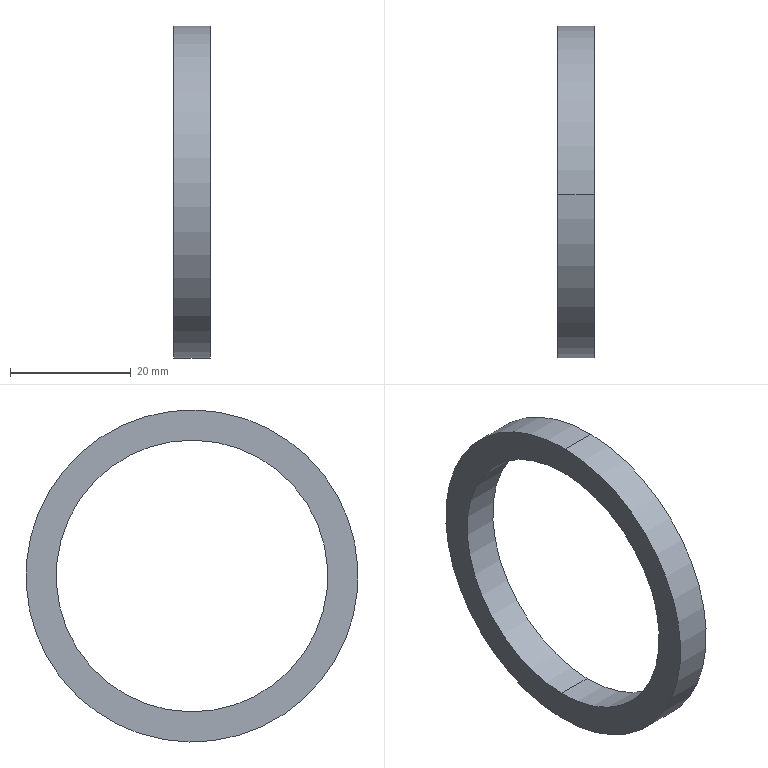Component | SolidWorks | 216InnerTubeAssembly-1_BearingSpacer1-1 | 1 solid | 6 faces | box 6 x 55 x 55 mm | volume 4712 mm3 | cylinder 4 | plane 2 | commonest cylinder face diameters 45 x2 55 x2 | material Alloy Steel
build123d program:
from build123d import *

# Parameters (mm, degrees)
MODEL_W = 5.999
MODEL_H = 5


with BuildPart() as part:
    # Model → Revolve1 (revolve)
    with BuildSketch(Plane.XY, mode=Mode.PRIVATE) as revolve1_sk:
        with Locations((2.999, 25)):
            Rectangle(MODEL_W, MODEL_H)
    revolve(revolve1_sk.sketch.rotate(Axis((0, 0, 0), (1, 0, 0)), 90), axis=Axis((0, 0, 0), (1, 0, 0)))


solid = part.part

# Placed as in the assembly
solid = solid.moved(Location((841.279, 0, 0), (0, 0, 0)))
STEP:
#1=COLOUR_RGB('',0.7922,0.8196,0.9333);
#2=FILL_AREA_STYLE_COLOUR('',#1);
#3=FILL_AREA_STYLE('',(#2));
#4=SURFACE_STYLE_FILL_AREA(#3);
#5=SURFACE_SIDE_STYLE('',(#4));
#6=SURFACE_STYLE_USAGE(.BOTH.,#5);
#7=PRESENTATION_STYLE_ASSIGNMENT((#6));
#8=CARTESIAN_POINT('',(33.357,0.01591,-0.8857));
#9=VERTEX_POINT('',#8);
#10=CARTESIAN_POINT('',(33.357,-0.01591,0.8857));
#11=VERTEX_POINT('',#10);
#12=CARTESIAN_POINT('',(33.357,-0.,0.));
#13=DIRECTION('',(-1.,-0.,0.));
#14=DIRECTION('',(0.,-0.01796,0.9998));
#15=AXIS2_PLACEMENT_3D('',#12,#13,#14);
#16=CIRCLE('',#15,0.8858);
#17=EDGE_CURVE('',#9,#11,#16,.T.);
#18=ORIENTED_EDGE('',*,*,#17,.F.);
#19=CARTESIAN_POINT('',(33.121,0.01591,-0.8857));
#20=VERTEX_POINT('',#19);
#21=CARTESIAN_POINT('',(33.121,0.01591,-0.8857));
#22=DIRECTION('',(-1.,-0.,0.));
#23=VECTOR('',#22,39.37);
#24=LINE('',#21,#23);
#25=EDGE_CURVE('',#9,#20,#24,.T.);
#26=ORIENTED_EDGE('',*,*,#25,.T.);
#27=CARTESIAN_POINT('',(33.121,-0.01591,0.8857));
#28=VERTEX_POINT('',#27);
#29=CARTESIAN_POINT('',(33.121,-0.,0.));
#30=DIRECTION('',(-1.,-0.,0.));
#31=DIRECTION('',(0.,-0.01796,0.9998));
#32=AXIS2_PLACEMENT_3D('',#29,#30,#31);
#33=CIRCLE('',#32,0.8858);
#34=EDGE_CURVE('',#20,#28,#33,.T.);
#35=ORIENTED_EDGE('',*,*,#34,.T.);
#36=CARTESIAN_POINT('',(33.121,-0.01591,0.8857));
#37=DIRECTION('',(-1.,-0.,0.));
#38=VECTOR('',#37,39.37);
#39=LINE('',#36,#38);
#40=EDGE_CURVE('',#11,#28,#39,.T.);
#41=ORIENTED_EDGE('',*,*,#40,.F.);
#42=EDGE_LOOP('',(#18,#26,#35,#41));
#43=FACE_OUTER_BOUND('',#42,.T.);
#44=CARTESIAN_POINT('',(33.121,-0.,0.));
#45=DIRECTION('',(-1.,-0.,0.));
#46=DIRECTION('',(0.,-0.01796,0.9998));
#47=AXIS2_PLACEMENT_3D('',#44,#45,#46);
#48=CYLINDRICAL_SURFACE('',#47,0.8858);
#49=ADVANCED_FACE('',(#43),#48,.F.);
#50=CARTESIAN_POINT('',(33.357,-0.01944,1.083));
#51=VERTEX_POINT('',#50);
#52=CARTESIAN_POINT('',(33.357,0.01944,-1.083));
#53=VERTEX_POINT('',#52);
#54=CARTESIAN_POINT('',(33.357,-0.,0.));
#55=DIRECTION('',(-1.,-0.,0.));
#56=DIRECTION('',(0.,-0.01796,0.9998));
#57=AXIS2_PLACEMENT_3D('',#54,#55,#56);
#58=CIRCLE('',#57,1.083);
#59=EDGE_CURVE('',#51,#53,#58,.T.);
#60=ORIENTED_EDGE('',*,*,#59,.T.);
#61=CARTESIAN_POINT('',(33.121,0.01944,-1.083));
#62=VERTEX_POINT('',#61);
#63=CARTESIAN_POINT('',(33.121,0.01944,-1.083));
#64=DIRECTION('',(-1.,-0.,0.));
#65=VECTOR('',#64,39.37);
#66=LINE('',#63,#65);
#67=EDGE_CURVE('',#53,#62,#66,.T.);
#68=ORIENTED_EDGE('',*,*,#67,.T.);
#69=CARTESIAN_POINT('',(33.121,-0.01944,1.083));
#70=VERTEX_POINT('',#69);
#71=CARTESIAN_POINT('',(33.121,-0.,0.));
#72=DIRECTION('',(-1.,-0.,0.));
#73=DIRECTION('',(0.,-0.01796,0.9998));
#74=AXIS2_PLACEMENT_3D('',#71,#72,#73);
#75=CIRCLE('',#74,1.083);
#76=EDGE_CURVE('',#70,#62,#75,.T.);
#77=ORIENTED_EDGE('',*,*,#76,.F.);
#78=CARTESIAN_POINT('',(33.121,-0.01944,1.083));
#79=DIRECTION('',(-1.,-0.,0.));
#80=VECTOR('',#79,39.37);
#81=LINE('',#78,#80);
#82=EDGE_CURVE('',#51,#70,#81,.T.);
#83=ORIENTED_EDGE('',*,*,#82,.F.);
#84=EDGE_LOOP('',(#60,#68,#77,#83));
#85=FACE_OUTER_BOUND('',#84,.T.);
#86=CARTESIAN_POINT('',(33.121,-0.,0.));
#87=DIRECTION('',(-1.,-0.,0.));
#88=DIRECTION('',(0.,-0.01796,0.9998));
#89=AXIS2_PLACEMENT_3D('',#86,#87,#88);
#90=CYLINDRICAL_SURFACE('',#89,1.083);
#91=ADVANCED_FACE('',(#85),#90,.T.);
#92=ORIENTED_EDGE('',*,*,#67,.F.);
#93=CARTESIAN_POINT('',(33.357,-0.,0.));
#94=DIRECTION('',(-1.,-0.,0.));
#95=DIRECTION('',(0.,-0.01796,0.9998));
#96=AXIS2_PLACEMENT_3D('',#93,#94,#95);
#97=CIRCLE('',#96,1.083);
#98=EDGE_CURVE('',#53,#51,#97,.T.);
#99=ORIENTED_EDGE('',*,*,#98,.T.);
#100=ORIENTED_EDGE('',*,*,#82,.T.);
#101=CARTESIAN_POINT('',(33.121,-0.,0.));
#102=DIRECTION('',(-1.,-0.,0.));
#103=DIRECTION('',(0.,-0.01796,0.9998));
#104=AXIS2_PLACEMENT_3D('',#101,#102,#103);
#105=CIRCLE('',#104,1.083);
#106=EDGE_CURVE('',#62,#70,#105,.T.);
#107=ORIENTED_EDGE('',*,*,#106,.F.);
#108=EDGE_LOOP('',(#92,#99,#100,#107));
#109=FACE_OUTER_BOUND('',#108,.T.);
#110=CARTESIAN_POINT('',(33.121,-0.,0.));
#111=DIRECTION('',(-1.,-0.,0.));
#112=DIRECTION('',(0.,-0.01796,0.9998));
#113=AXIS2_PLACEMENT_3D('',#110,#111,#112);
#114=CYLINDRICAL_SURFACE('',#113,1.083);
#115=ADVANCED_FACE('',(#109),#114,.T.);
#116=CARTESIAN_POINT('',(33.121,-0.,0.));
#117=DIRECTION('',(-1.,-0.,0.));
#118=DIRECTION('',(0.,-0.01796,0.9998));
#119=AXIS2_PLACEMENT_3D('',#116,#117,#118);
#120=CIRCLE('',#119,0.8858);
#121=EDGE_CURVE('',#28,#20,#120,.T.);
#122=ORIENTED_EDGE('',*,*,#121,.F.);
#123=ORIENTED_EDGE('',*,*,#34,.F.);
#124=EDGE_LOOP('',(#122,#123));
#125=FACE_BOUND('',#124,.T.);
#126=ORIENTED_EDGE('',*,*,#76,.T.);
#127=ORIENTED_EDGE('',*,*,#106,.T.);
#128=EDGE_LOOP('',(#126,#127));
#129=FACE_OUTER_BOUND('',#128,.T.);
#130=CARTESIAN_POINT('',(33.121,1.083,0.01944));
#131=DIRECTION('',(1.,0.,-0.));
#132=DIRECTION('',(-0.,0.01796,-0.9998));
#133=AXIS2_PLACEMENT_3D('',#130,#131,#132);
#134=PLANE('',#133);
#135=ADVANCED_FACE('',(#125,#129),#134,.F.);
#136=ORIENTED_EDGE('',*,*,#25,.F.);
#137=CARTESIAN_POINT('',(33.357,-0.,0.));
#138=DIRECTION('',(-1.,-0.,0.));
#139=DIRECTION('',(0.,-0.01796,0.9998));
#140=AXIS2_PLACEMENT_3D('',#137,#138,#139);
#141=CIRCLE('',#140,0.8858);
#142=EDGE_CURVE('',#11,#9,#141,.T.);
#143=ORIENTED_EDGE('',*,*,#142,.F.);
#144=ORIENTED_EDGE('',*,*,#40,.T.);
#145=ORIENTED_EDGE('',*,*,#121,.T.);
#146=EDGE_LOOP('',(#136,#143,#144,#145));
#147=FACE_OUTER_BOUND('',#146,.T.);
#148=CARTESIAN_POINT('',(33.121,-0.,0.));
#149=DIRECTION('',(-1.,-0.,0.));
#150=DIRECTION('',(0.,-0.01796,0.9998));
#151=AXIS2_PLACEMENT_3D('',#148,#149,#150);
#152=CYLINDRICAL_SURFACE('',#151,0.8858);
#153=ADVANCED_FACE('',(#147),#152,.F.);
#154=ORIENTED_EDGE('',*,*,#59,.F.);
#155=ORIENTED_EDGE('',*,*,#98,.F.);
#156=EDGE_LOOP('',(#154,#155));
#157=FACE_OUTER_BOUND('',#156,.T.);
#158=ORIENTED_EDGE('',*,*,#142,.T.);
#159=ORIENTED_EDGE('',*,*,#17,.T.);
#160=EDGE_LOOP('',(#158,#159));
#161=FACE_BOUND('',#160,.T.);
#162=CARTESIAN_POINT('',(33.357,0.8857,0.01591));
#163=DIRECTION('',(-1.,-0.,0.));
#164=DIRECTION('',(0.,-0.01796,0.9998));
#165=AXIS2_PLACEMENT_3D('',#162,#163,#164);
#166=PLANE('',#165);
#167=ADVANCED_FACE('',(#157,#161),#166,.F.);
#168=CLOSED_SHELL('',(#49,#91,#115,#135,#153,#167));
#169=MANIFOLD_SOLID_BREP('',#168);
#170=STYLED_ITEM('',(#7),#169);
#171=(LENGTH_UNIT()NAMED_UNIT(*)SI_UNIT($,.METRE.));
#172=LENGTH_MEASURE_WITH_UNIT(LENGTH_MEASURE(0.0254),#171);
#173=DIMENSIONAL_EXPONENTS(1.,0.,0.,0.,0.,0.,0.);
#174=(CONVERSION_BASED_UNIT('',#172)LENGTH_UNIT()NAMED_UNIT(#173));
#175=UNCERTAINTY_MEASURE_WITH_UNIT(LENGTH_MEASURE(0.00001),#174,'','');
#176=(NAMED_UNIT(*)PLANE_ANGLE_UNIT()SI_UNIT($,.RADIAN.));
#177=(NAMED_UNIT(*)SI_UNIT($,.STERADIAN.)SOLID_ANGLE_UNIT());
#178=(GEOMETRIC_REPRESENTATION_CONTEXT(3)GLOBAL_UNCERTAINTY_ASSIGNED_CONTEXT((#175))GLOBAL_UNIT_ASSIGNED_CONTEXT((#174,#176,#177))REPRESENTATION_CONTEXT('',''));
#179=MECHANICAL_DESIGN_GEOMETRIC_PRESENTATION_REPRESENTATION('',(#170),#178);
#180=CARTESIAN_POINT('',(0.,0.,0.));
#181=DIRECTION('',(0.,0.,1.));
#182=DIRECTION('',(1.,0.,0.));
#183=AXIS2_PLACEMENT_3D('',#180,#181,#182);
#184=(LENGTH_UNIT()NAMED_UNIT(*)SI_UNIT($,.METRE.));
#185=LENGTH_MEASURE_WITH_UNIT(LENGTH_MEASURE(0.0254),#184);
#186=DIMENSIONAL_EXPONENTS(1.,0.,0.,0.,0.,0.,0.);
#187=(CONVERSION_BASED_UNIT('',#185)LENGTH_UNIT()NAMED_UNIT(#186));
#188=UNCERTAINTY_MEASURE_WITH_UNIT(LENGTH_MEASURE(0.00001),#187,'','');
#189=(NAMED_UNIT(*)PLANE_ANGLE_UNIT()SI_UNIT($,.RADIAN.));
#190=(NAMED_UNIT(*)SI_UNIT($,.STERADIAN.)SOLID_ANGLE_UNIT());
#191=(GEOMETRIC_REPRESENTATION_CONTEXT(3)GLOBAL_UNCERTAINTY_ASSIGNED_CONTEXT((#188))GLOBAL_UNIT_ASSIGNED_CONTEXT((#187,#189,#190))REPRESENTATION_CONTEXT('',''));
#192=ADVANCED_BREP_SHAPE_REPRESENTATION('',(#169,#183),#191);
#193=PRESENTATION_LAYER_ASSIGNMENT('','',(#170));